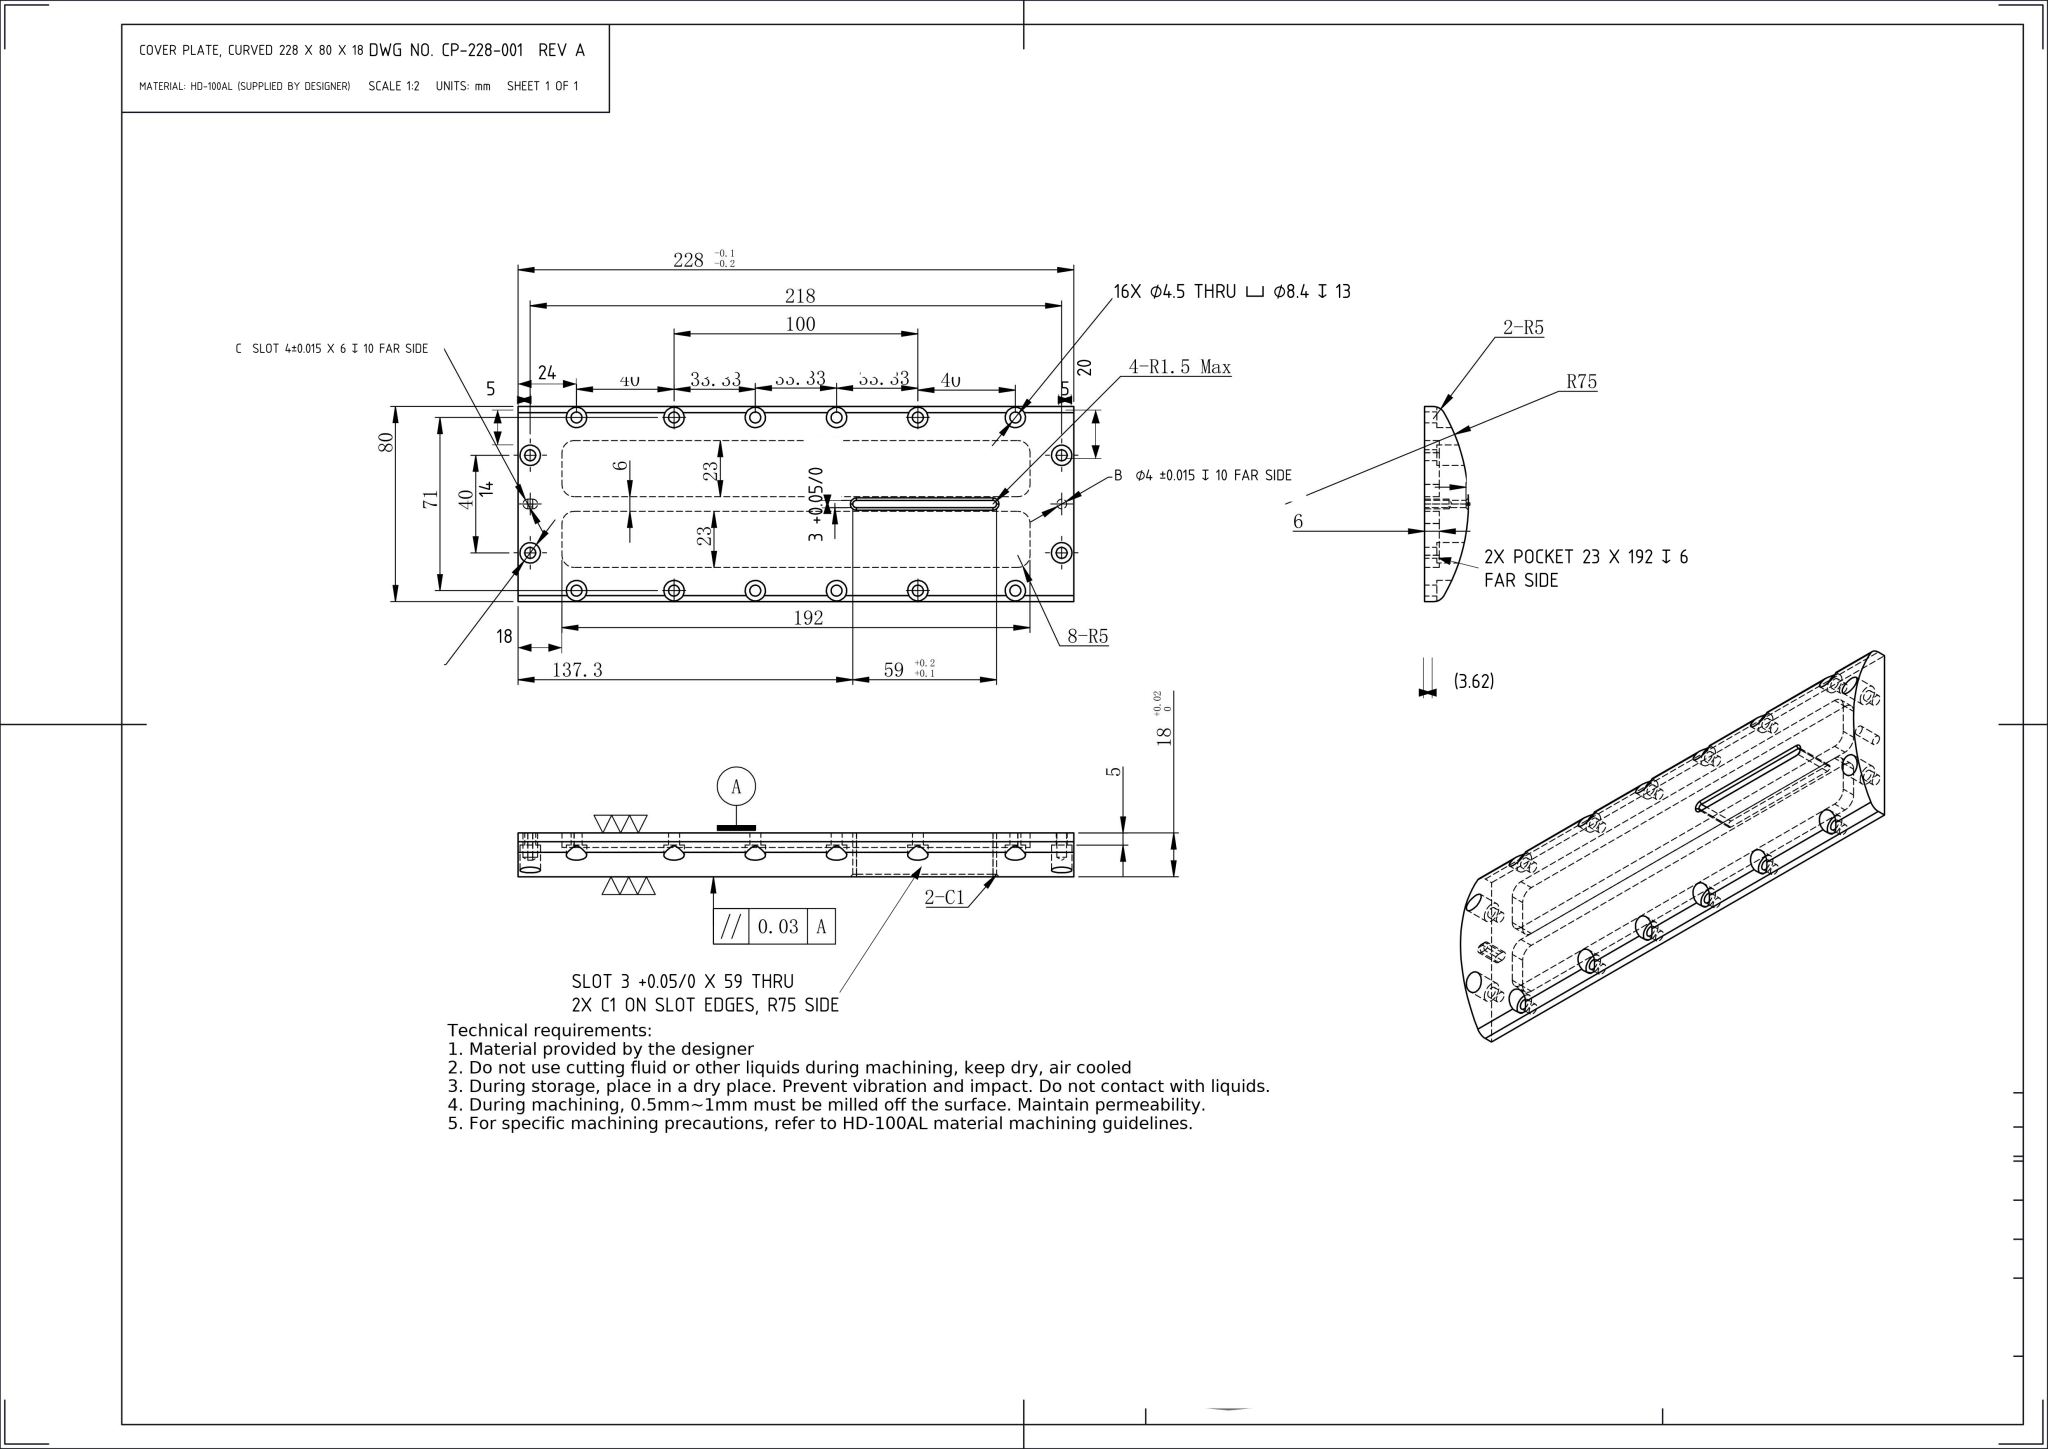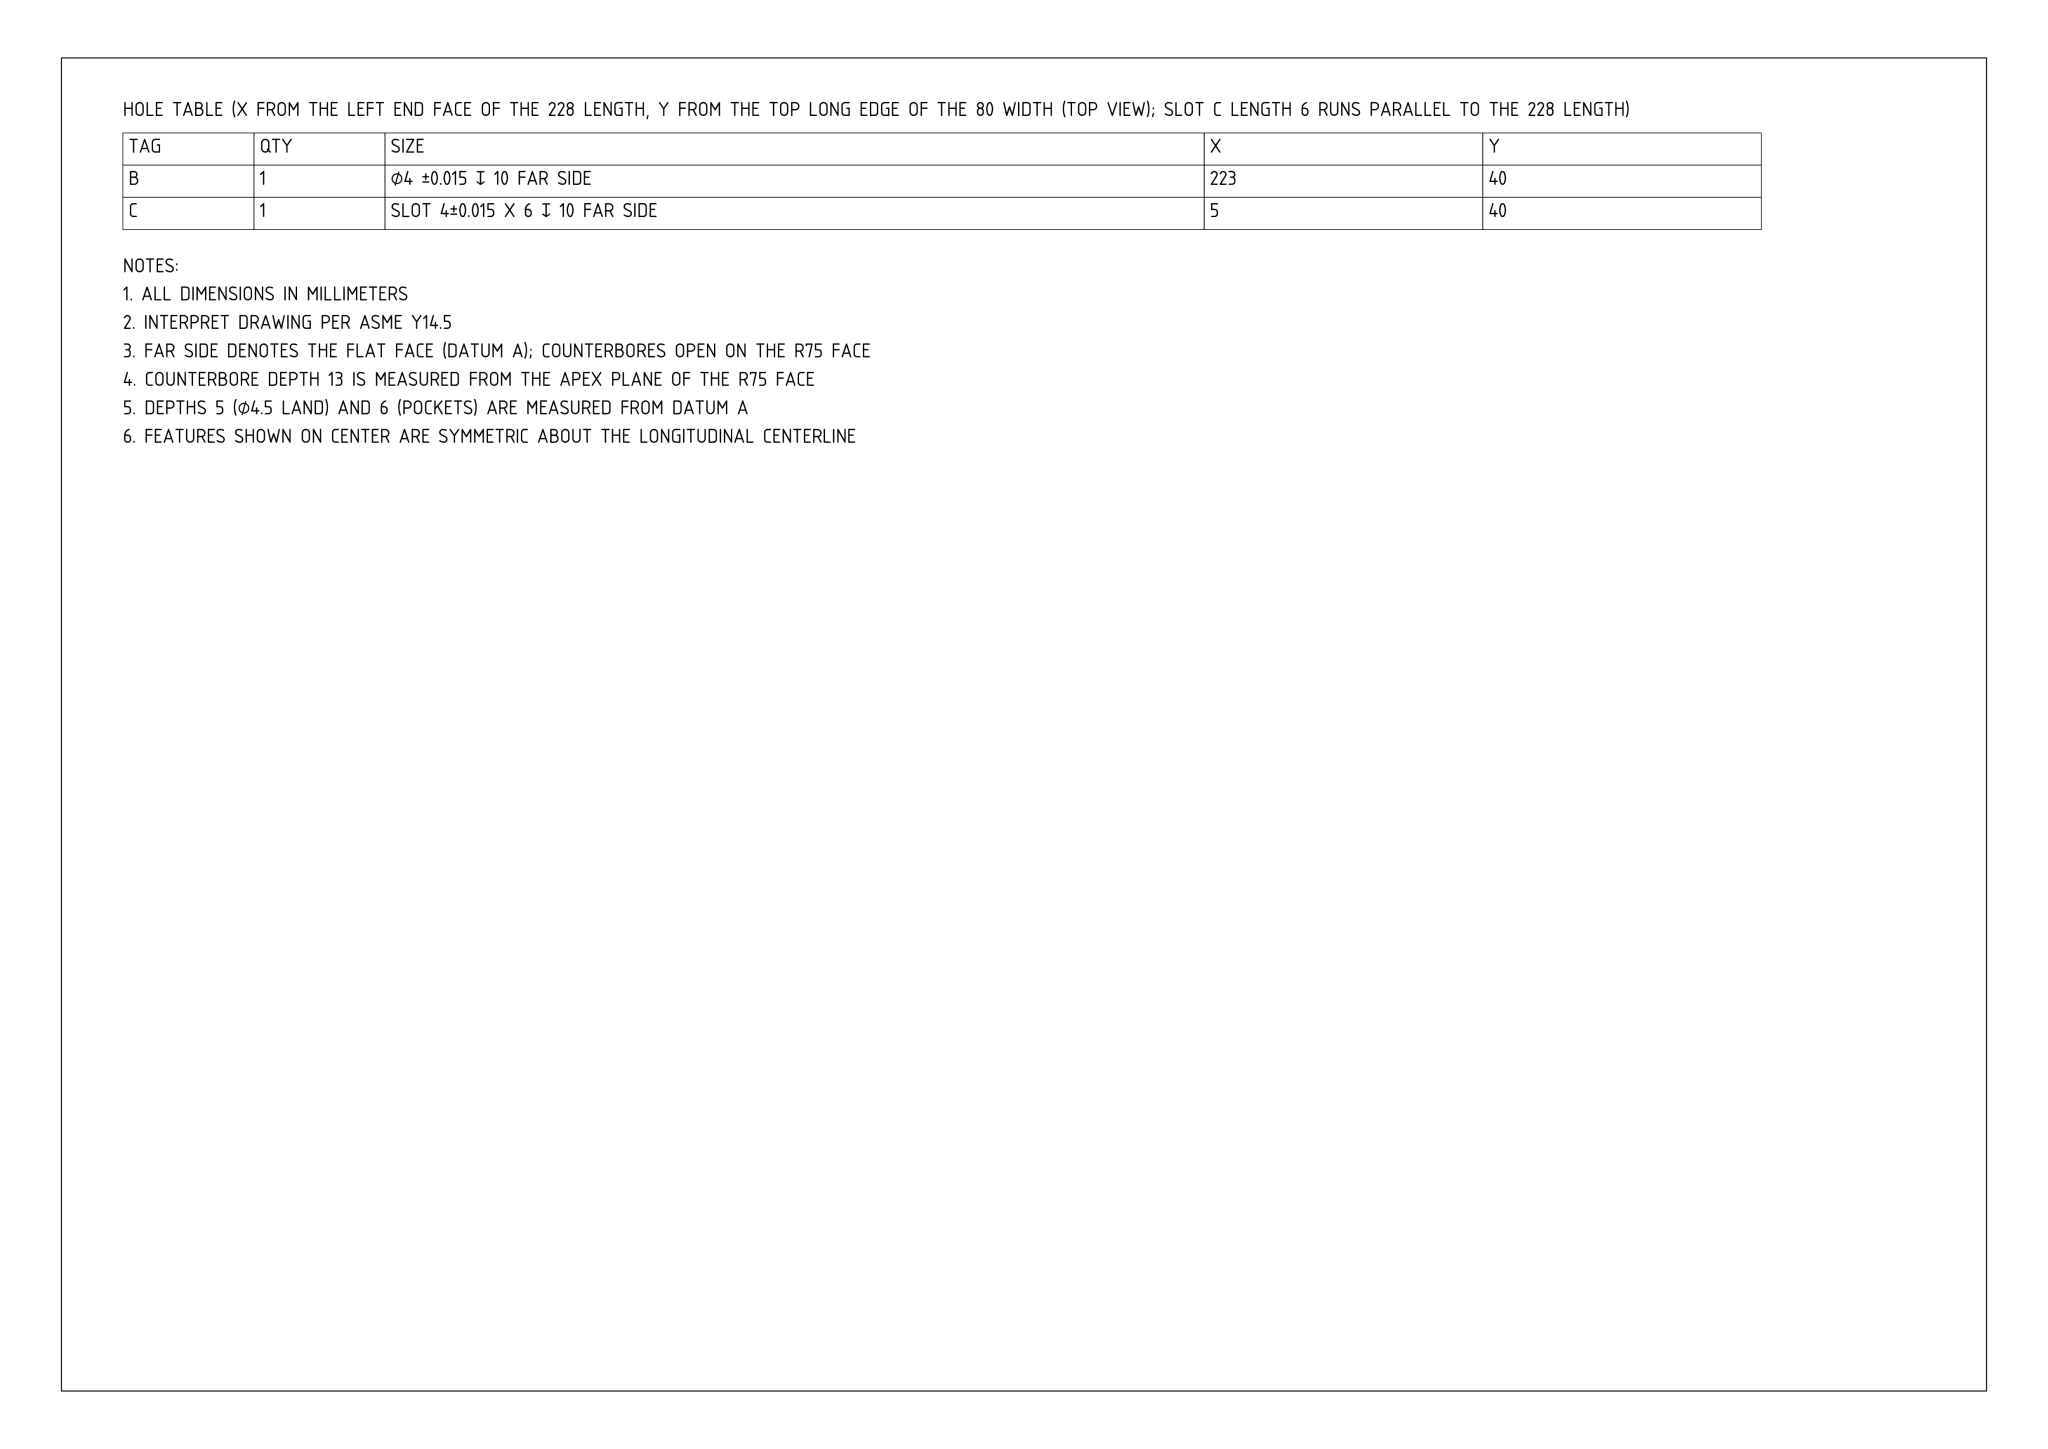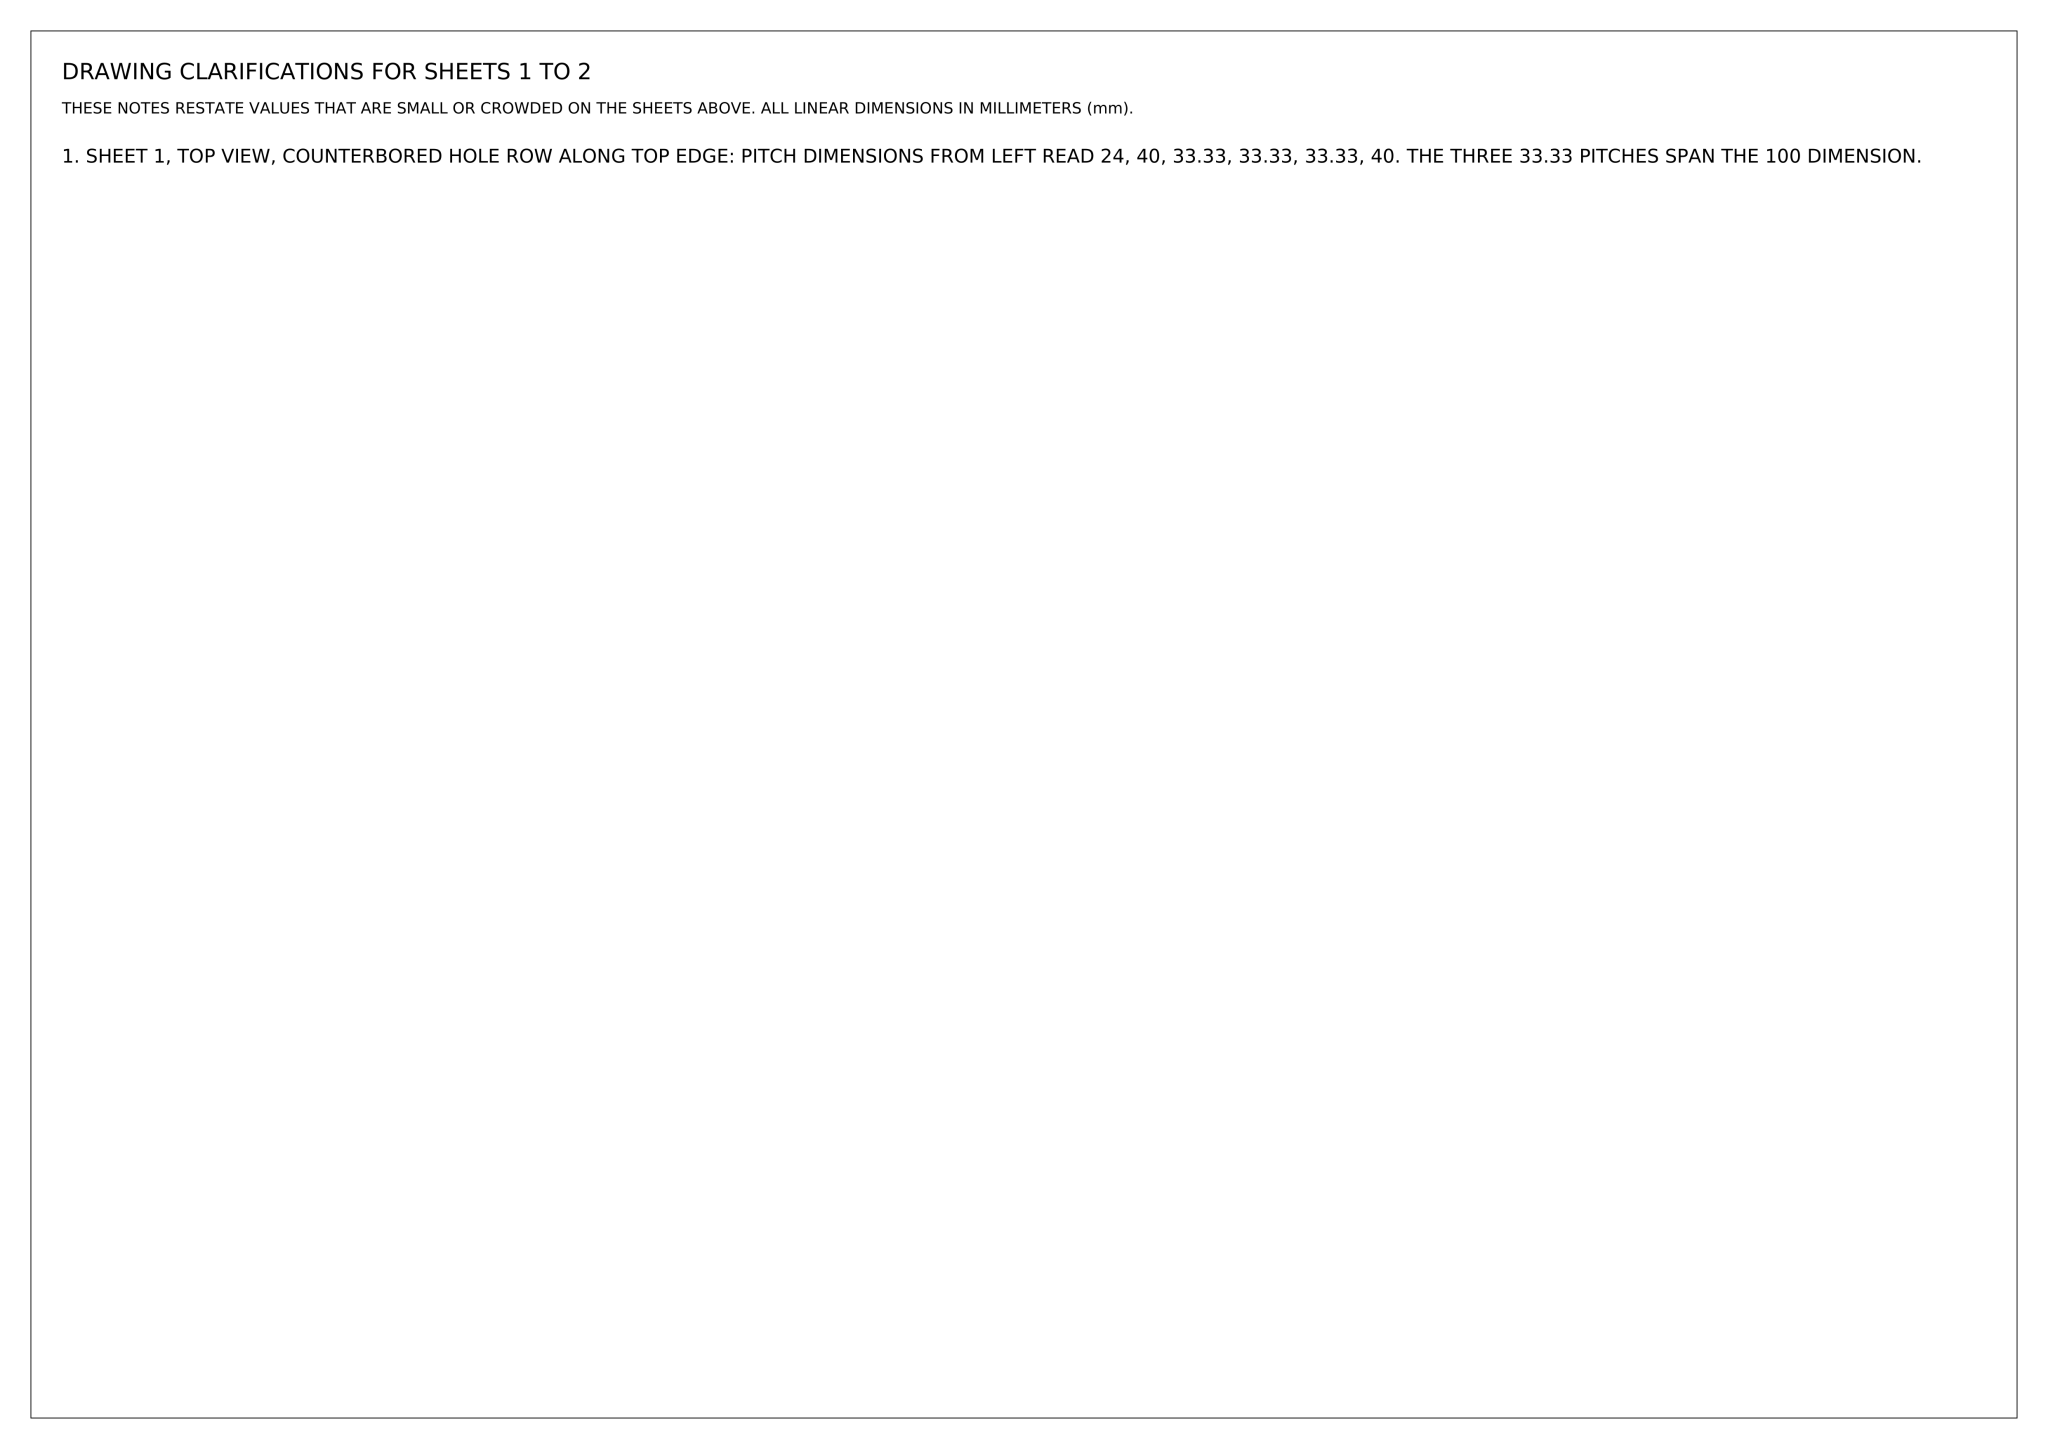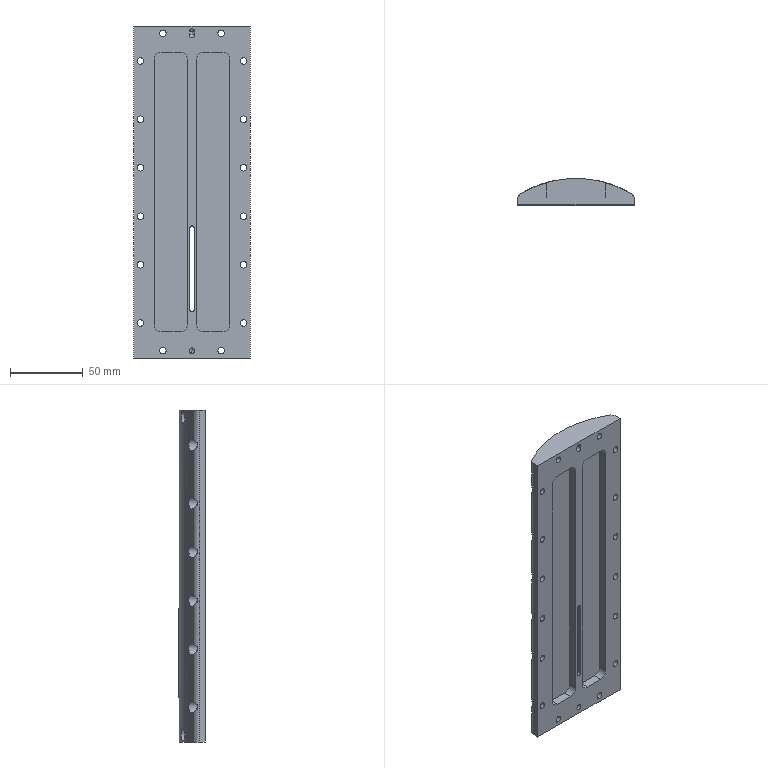Part | NX | mm | 1 solid | 132 faces | box 80 x 18 x 228 mm | volume 197302 mm3 | cylinder 84 | plane 39 | cone 5 | spline 4 | commonest cylinder face diameters 8.4 x32 4.5 x32 10 x10 4 x5 3 x4 150 x1